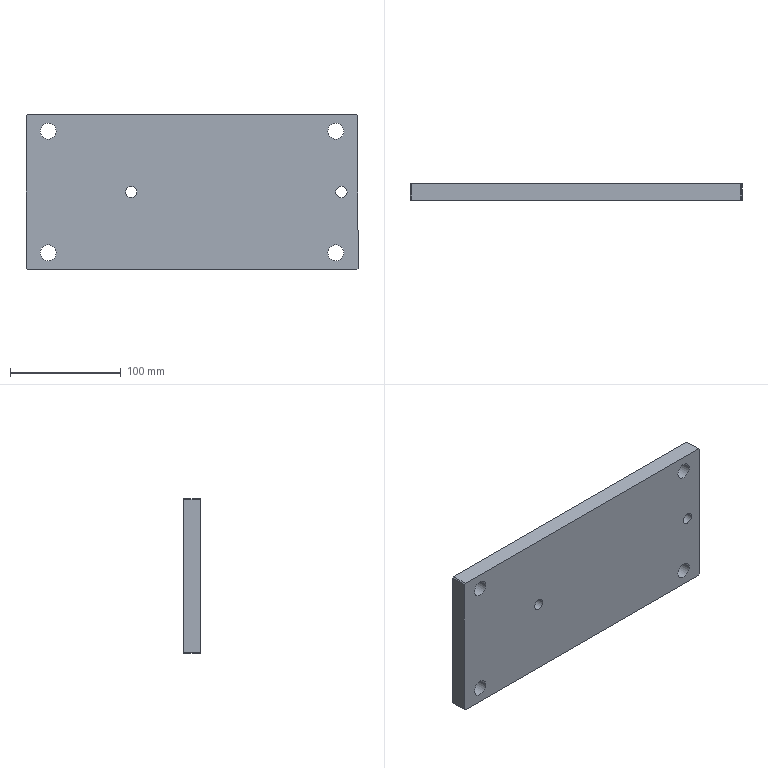Component | SolidWorks | AdjustmentFrameBasePlate9.26-1 | 1 solid | 22 faces | box 300 x 15 x 140 mm | volume 617611 mm3 | cylinder 12 | plane 10 | commonest cylinder face diameters 14.5 x8 10.2 x4 | material AISI 1045 Steel, Cold Drawn
build123d program:
from build123d import *

# Parameters (mm, degrees)
SKETCH1_W           = 300
SKETCH1_H           = 140
BOSS_EXTRUDE1_DEPTH = 15
SKETCH2_R           = 7.25
CUT_EXTRUDE1_DEPTH  = 332.399
M12_TAPPED_HOLE1_D  = 10.2
CHAMFER1_SIZE       = 1


with BuildPart() as part:
    # Sketch1 → Boss-Extrude1 (new body)
    with BuildSketch(Plane.XY):
        with Locations((150, -70)):
            Rectangle(SKETCH1_W, SKETCH1_H)
    extrude(amount=BOSS_EXTRUDE1_DEPTH)

    # Sketch2 → Cut-Extrude1 (cut, through all)
    with BuildSketch(Plane(origin=(0, 0, 0), x_dir=(-1, 0, 0), z_dir=(0, 0, -1))):
        with Locations((-280, -15)):
            Circle(SKETCH2_R)
        with Locations(Location((-20, -15, 0), (0, 0, 180))):
            Circle(SKETCH2_R)
        with Locations((-20, -125)):
            Circle(SKETCH2_R)
        with Locations(Location((-280, -125, 0), (0, 0, 180))):
            Circle(SKETCH2_R)
    extrude(amount=-CUT_EXTRUDE1_DEPTH, mode=Mode.SUBTRACT)

    # M12 Tapped Hole1 (through all)
    with Locations(Plane(origin=(0, 0, 0), x_dir=(-1, 0, 0), z_dir=(0, 0, -1))):
        with Locations((-285, -70), (-95, -70)):
            Hole(M12_TAPPED_HOLE1_D / 2)

    # Chamfer1
    chamfer1_edges = [part.edges().sort_by_distance(p)[0] for p in [
        (0, 0, 7.5),
        (300, 0, 7.5),
        (300, -140, 7.5),
        (0, -140, 7.5),
    ]]
    chamfer(chamfer1_edges, length=CHAMFER1_SIZE)


solid = part.part

# Placed as in the assembly
solid = solid.moved(Location((13.705, -283, 85.25), (90, 0, 0)))